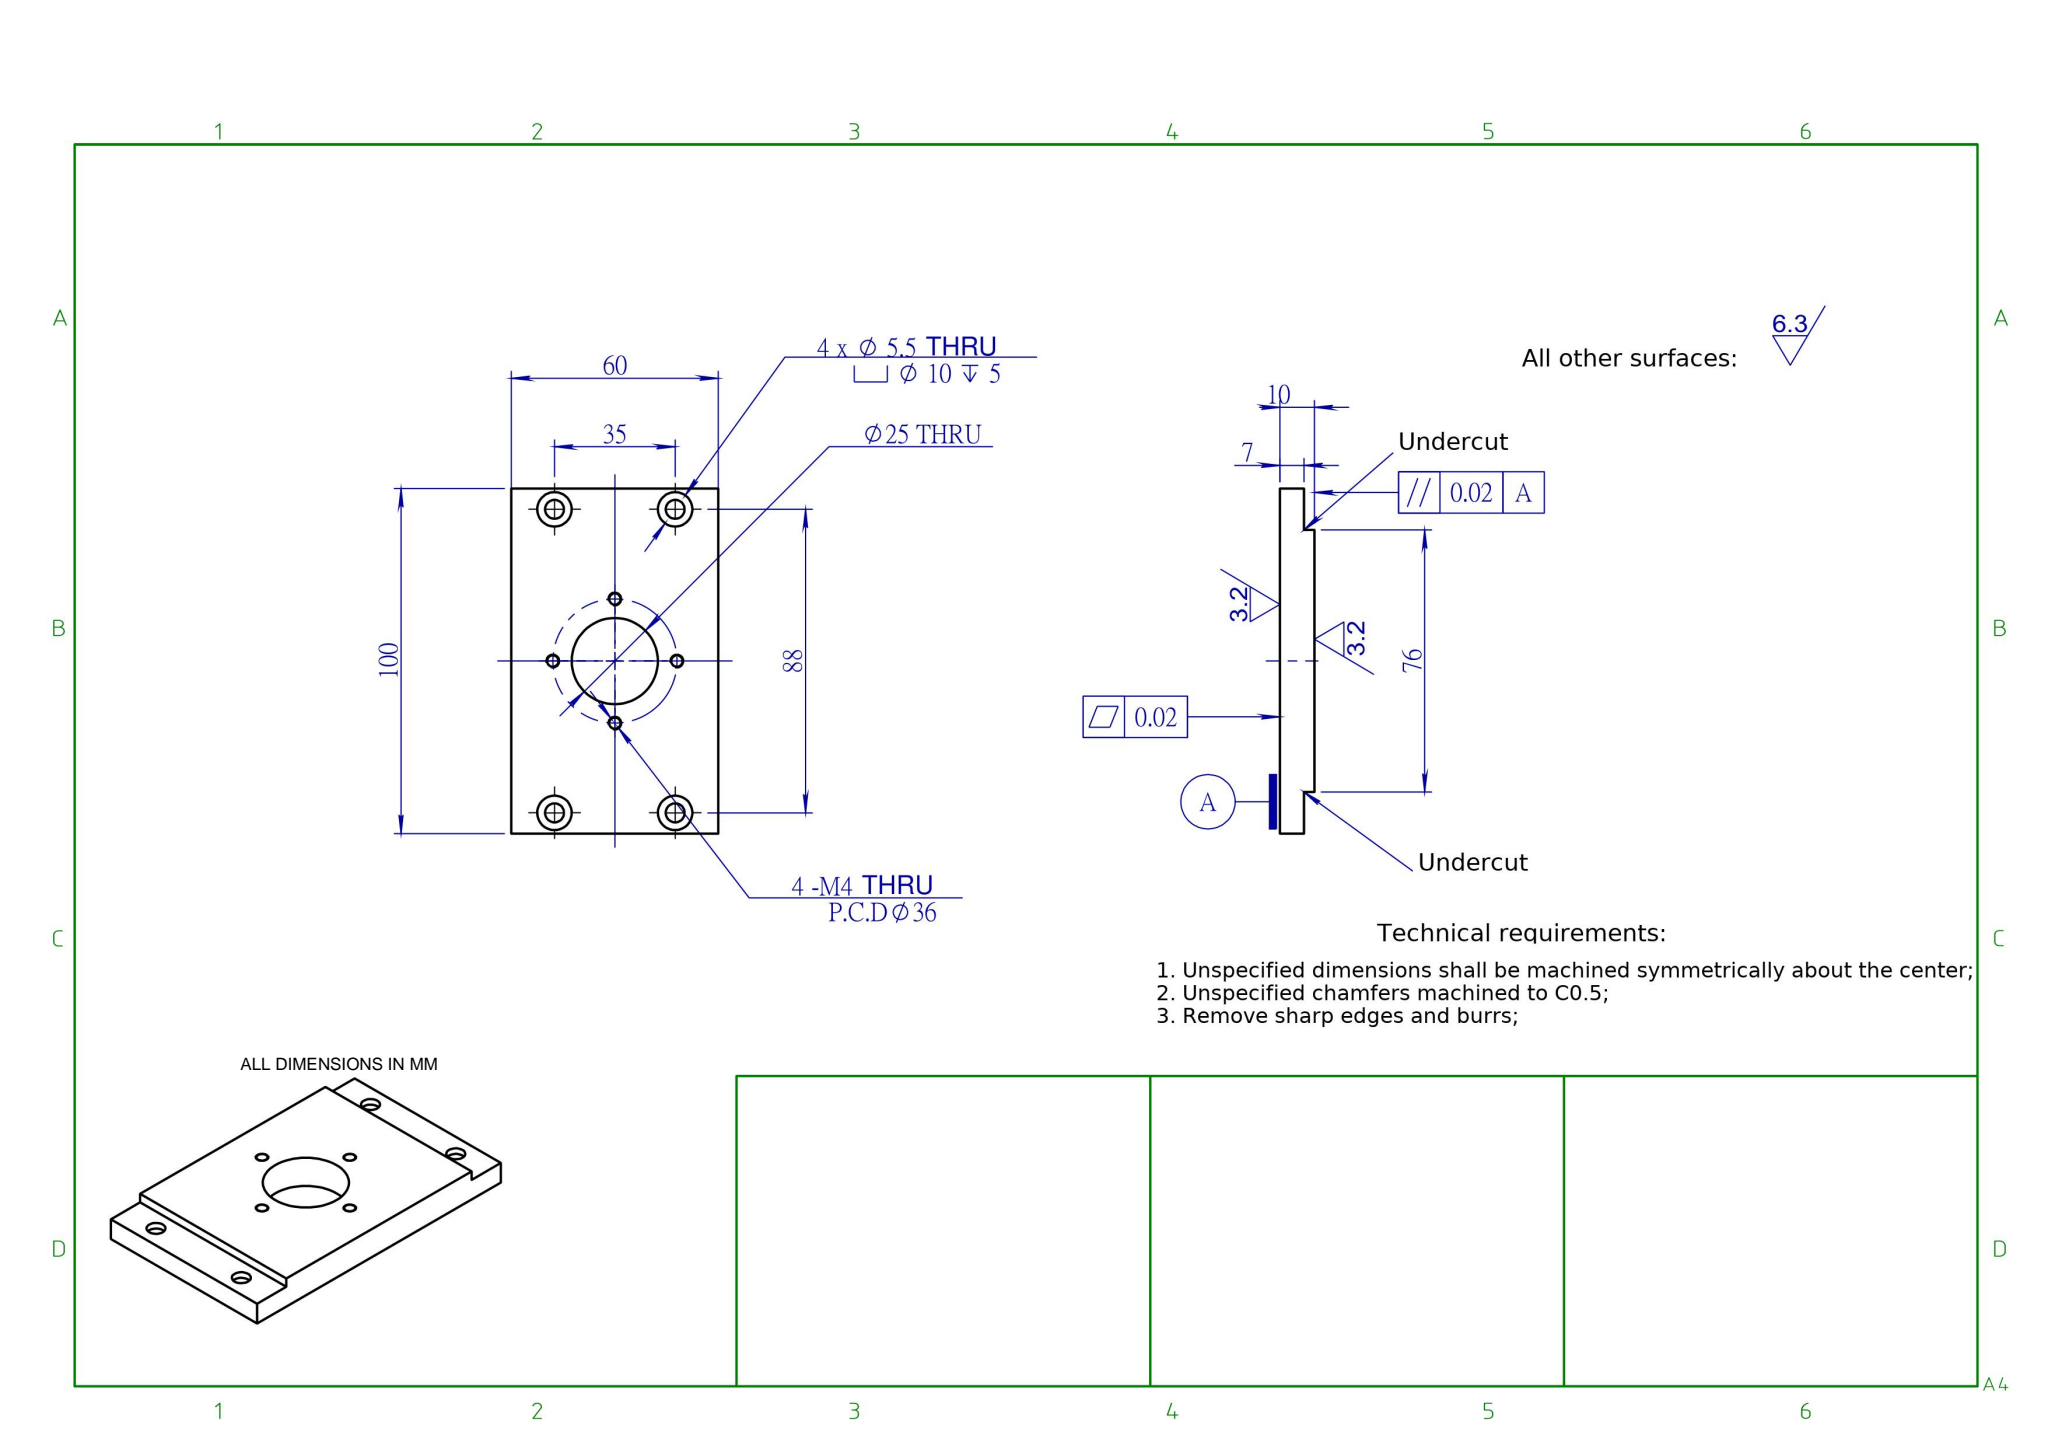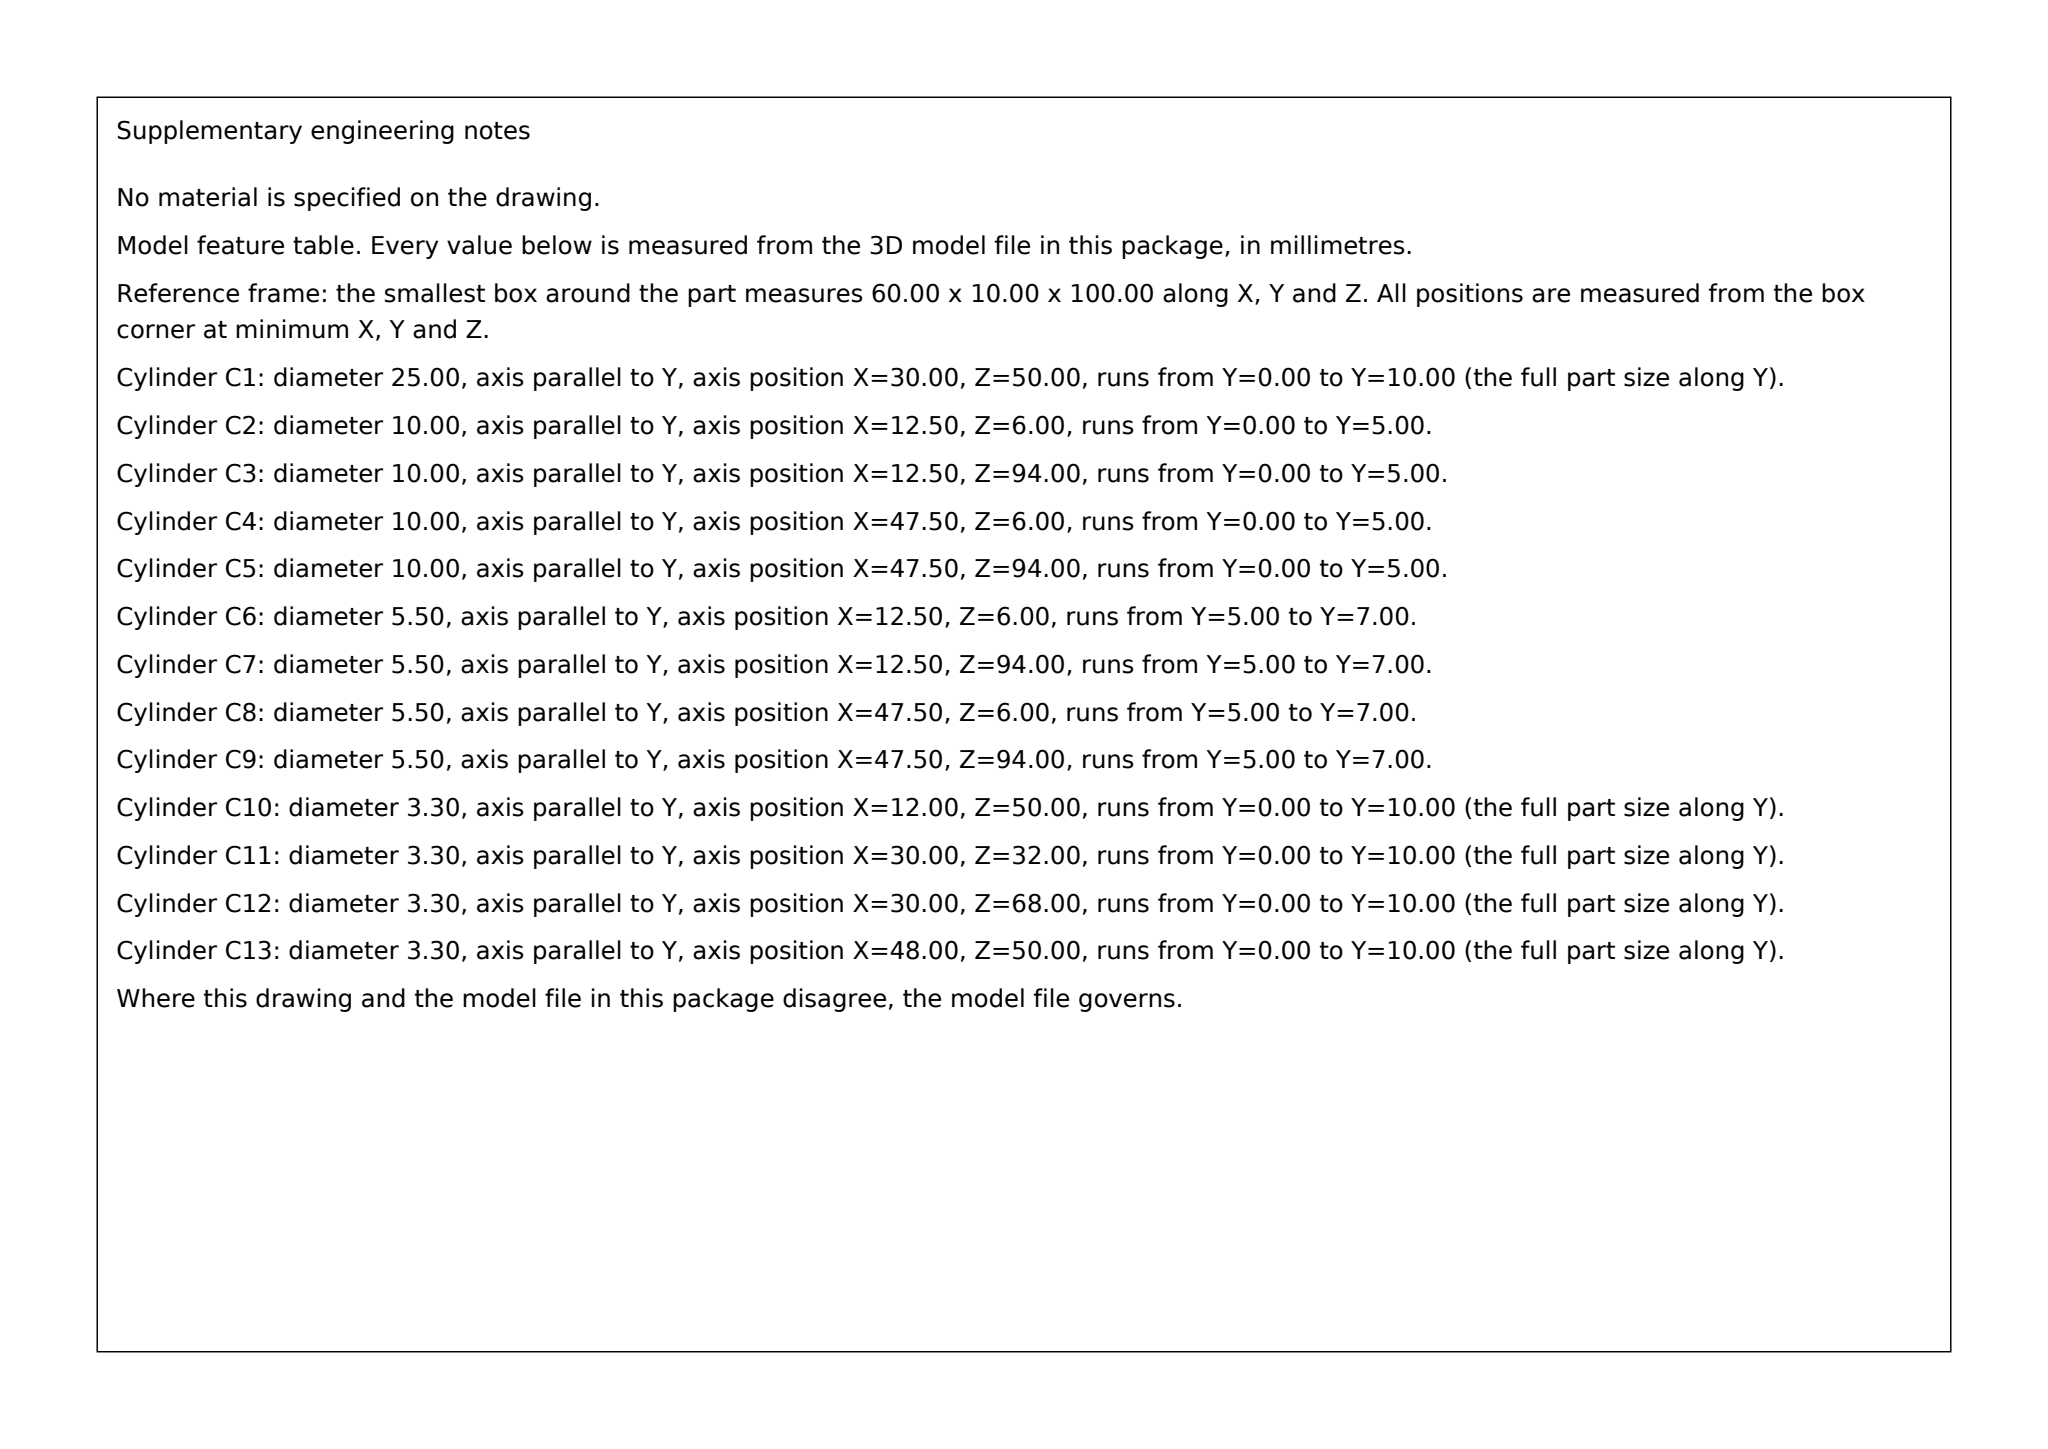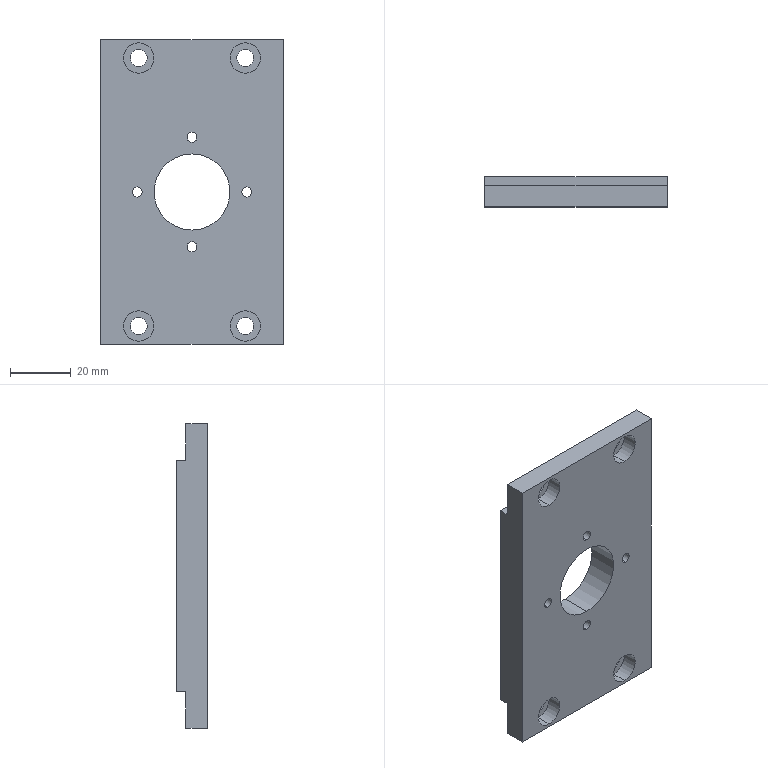Part | SolidWorks | mm | 1 solid | 40 faces | box 60 x 10 x 100 mm | volume 48668 mm3 | cylinder 26 | plane 14 | commonest cylinder face diameters 3.3 x8 10 x8 5.5 x8 25 x2
build123d program:
from build123d import *

# Parameters (mm, degrees)
SKETCH1_W                                            = 100
SKETCH1_H                                            = 10
EXTRUDE1_DEPTH                                       = 60
SKETCH2_R                                            = 12.5
CUT_EXTRUDE1_DEPTH                                   = 118.047
M5_HEX_SOCKET_HEAD_CAP_SCREW_COUNTERBORE_D           = 5.5
M5_HEX_SOCKET_HEAD_CAP_SCREW_COUNTERBORE_CBORE_D     = 10
M5_HEX_SOCKET_HEAD_CAP_SCREW_COUNTERBORE_CBORE_DEPTH = 5
SKETCH12_W                                           = 60
SKETCH12_H                                           = 12
CUT_EXTRUDE2_DEPTH                                   = 3
M4_TAPPED_HOLE3_D                                    = 3.3


with BuildPart() as part:
    # Sketch1 → Extrude1 (new body)
    with BuildSketch(Plane(origin=(0, 0, 0), x_dir=(0, 0, -1), z_dir=(1, 0, 0))):
        with Locations((50, -5)):
            Rectangle(SKETCH1_W, SKETCH1_H)
    extrude(amount=EXTRUDE1_DEPTH)

    # Sketch2 → Cut-Extrude1 (cut, through all)
    with BuildSketch(Plane(origin=(0, 0, 0), x_dir=(1, 0, 0), z_dir=(0, 1, 0))):
        with Locations(Location((30, 50, 0), (0, 0, 270))):
            Circle(SKETCH2_R)
    extrude(amount=-CUT_EXTRUDE1_DEPTH, mode=Mode.SUBTRACT)

    # M5 Hex Socket Head Cap Screw Counterbore (through all)
    with Locations(Plane.XZ.offset(10)):
        with Locations((12.5, -6), (47.5, -6), (47.5, -94), (12.5, -94)):
            CounterBoreHole(M5_HEX_SOCKET_HEAD_CAP_SCREW_COUNTERBORE_D / 2, M5_HEX_SOCKET_HEAD_CAP_SCREW_COUNTERBORE_CBORE_D / 2, M5_HEX_SOCKET_HEAD_CAP_SCREW_COUNTERBORE_CBORE_DEPTH)

    # Sketch12 → Cut-Extrude2 (cut)
    with BuildSketch(Plane(origin=(0, 0, 0), x_dir=(1, 0, 0), z_dir=(0, 1, 0))):
        with Locations((30, 94)):
            Rectangle(SKETCH12_W, SKETCH12_H)
        with Locations((30, 6)):
            Rectangle(SKETCH12_W, SKETCH12_H)
    extrude(amount=-CUT_EXTRUDE2_DEPTH, mode=Mode.SUBTRACT)

    # M4 Tapped Hole3 (through all)
    with Locations(Plane(origin=(0, 0, 0), x_dir=(-1, 0, 0), z_dir=(0, 1, 0))):
        with Locations((-12, -50), (-30, -32), (-48, -50), (-30, -68)):
            Hole(M4_TAPPED_HOLE3_D / 2)


solid = part.part